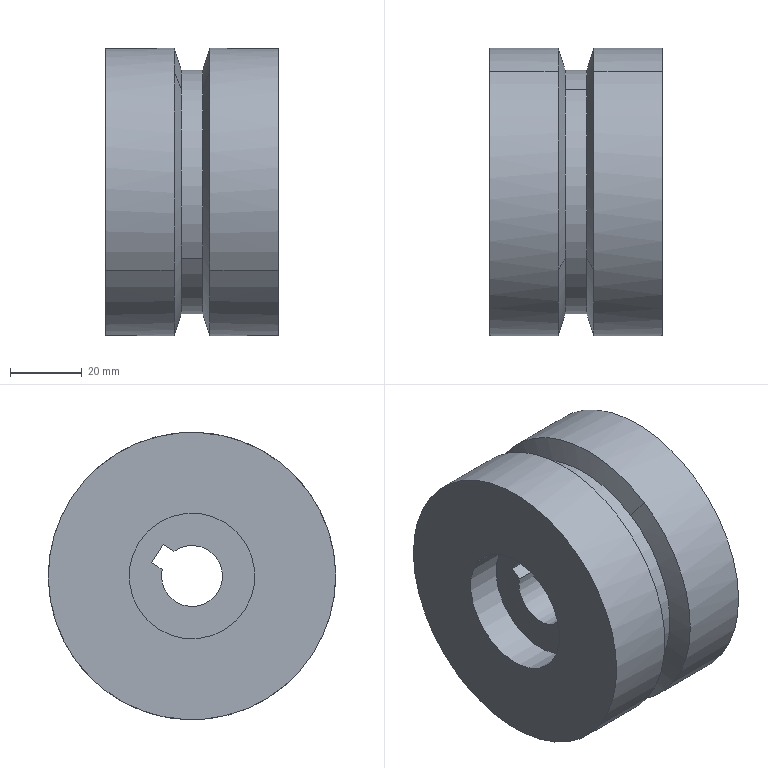Component | SolidWorks | CCD06DriveWheel-1 | 1 solid | 22 faces | box 48 x 80 x 80 mm | volume 203908 mm3 | cylinder 11 | plane 7 | cone 4 | commonest cylinder face diameters 35 x4 80 x4 68 x2 17 x1
STEP:
#1=COLOUR_RGB('',0.7922,0.8196,0.9333);
#2=FILL_AREA_STYLE_COLOUR('',#1);
#3=FILL_AREA_STYLE('',(#2));
#4=SURFACE_STYLE_FILL_AREA(#3);
#5=SURFACE_SIDE_STYLE('',(#4));
#6=SURFACE_STYLE_USAGE(.BOTH.,#5);
#7=PRESENTATION_STYLE_ASSIGNMENT((#6));
#8=CARTESIAN_POINT('',(-13.548,3.645,-4.274));
#9=VERTEX_POINT('',#8);
#10=CARTESIAN_POINT('',(-13.548,4.8,-3.522));
#11=VERTEX_POINT('',#10);
#12=CARTESIAN_POINT('',(-13.548,4.222,-3.898));
#13=DIRECTION('',(-1.,-0.,0.));
#14=DIRECTION('',(0.,0.8379,0.5458));
#15=AXIS2_PLACEMENT_3D('',#12,#13,#14);
#16=CIRCLE('',#15,0.689);
#17=EDGE_CURVE('',#9,#11,#16,.T.);
#18=ORIENTED_EDGE('',*,*,#17,.F.);
#19=CARTESIAN_POINT('',(-13.942,3.645,-4.274));
#20=VERTEX_POINT('',#19);
#21=CARTESIAN_POINT('',(-13.548,3.645,-4.274));
#22=DIRECTION('',(-1.,-0.,0.));
#23=VECTOR('',#22,39.37);
#24=LINE('',#21,#23);
#25=EDGE_CURVE('',#9,#20,#24,.T.);
#26=ORIENTED_EDGE('',*,*,#25,.T.);
#27=CARTESIAN_POINT('',(-13.942,4.8,-3.522));
#28=VERTEX_POINT('',#27);
#29=CARTESIAN_POINT('',(-13.942,4.222,-3.898));
#30=DIRECTION('',(-1.,-0.,0.));
#31=DIRECTION('',(0.,0.8379,0.5458));
#32=AXIS2_PLACEMENT_3D('',#29,#30,#31);
#33=CIRCLE('',#32,0.689);
#34=EDGE_CURVE('',#20,#28,#33,.T.);
#35=ORIENTED_EDGE('',*,*,#34,.T.);
#36=CARTESIAN_POINT('',(-13.548,4.8,-3.522));
#37=DIRECTION('',(-1.,-0.,0.));
#38=VECTOR('',#37,39.37);
#39=LINE('',#36,#38);
#40=EDGE_CURVE('',#11,#28,#39,.T.);
#41=ORIENTED_EDGE('',*,*,#40,.F.);
#42=EDGE_LOOP('',(#18,#26,#35,#41));
#43=FACE_OUTER_BOUND('',#42,.T.);
#44=CARTESIAN_POINT('',(-13.548,4.222,-3.898));
#45=DIRECTION('',(-1.,-0.,0.));
#46=DIRECTION('',(0.,0.8379,0.5458));
#47=AXIS2_PLACEMENT_3D('',#44,#45,#46);
#48=CYLINDRICAL_SURFACE('',#47,0.689);
#49=ADVANCED_FACE('',(#43),#48,.F.);
#50=CARTESIAN_POINT('',(-12.446,4.8,-3.522));
#51=VERTEX_POINT('',#50);
#52=CARTESIAN_POINT('',(-12.446,3.645,-4.274));
#53=VERTEX_POINT('',#52);
#54=CARTESIAN_POINT('',(-12.446,4.222,-3.898));
#55=DIRECTION('',(1.,0.,-0.));
#56=DIRECTION('',(-0.,-0.8379,-0.5458));
#57=AXIS2_PLACEMENT_3D('',#54,#55,#56);
#58=CIRCLE('',#57,0.689);
#59=EDGE_CURVE('',#51,#53,#58,.T.);
#60=ORIENTED_EDGE('',*,*,#59,.F.);
#61=CARTESIAN_POINT('',(-12.052,4.8,-3.522));
#62=VERTEX_POINT('',#61);
#63=CARTESIAN_POINT('',(-12.446,4.8,-3.522));
#64=DIRECTION('',(1.,0.,-0.));
#65=VECTOR('',#64,39.37);
#66=LINE('',#63,#65);
#67=EDGE_CURVE('',#51,#62,#66,.T.);
#68=ORIENTED_EDGE('',*,*,#67,.T.);
#69=CARTESIAN_POINT('',(-12.052,3.645,-4.274));
#70=VERTEX_POINT('',#69);
#71=CARTESIAN_POINT('',(-12.052,4.222,-3.898));
#72=DIRECTION('',(1.,0.,-0.));
#73=DIRECTION('',(-0.,-0.8379,-0.5458));
#74=AXIS2_PLACEMENT_3D('',#71,#72,#73);
#75=CIRCLE('',#74,0.689);
#76=EDGE_CURVE('',#62,#70,#75,.T.);
#77=ORIENTED_EDGE('',*,*,#76,.T.);
#78=CARTESIAN_POINT('',(-12.446,3.645,-4.274));
#79=DIRECTION('',(1.,0.,-0.));
#80=VECTOR('',#79,39.37);
#81=LINE('',#78,#80);
#82=EDGE_CURVE('',#53,#70,#81,.T.);
#83=ORIENTED_EDGE('',*,*,#82,.F.);
#84=EDGE_LOOP('',(#60,#68,#77,#83));
#85=FACE_OUTER_BOUND('',#84,.T.);
#86=CARTESIAN_POINT('',(-12.446,4.222,-3.898));
#87=DIRECTION('',(1.,0.,-0.));
#88=DIRECTION('',(-0.,-0.8379,-0.5458));
#89=AXIS2_PLACEMENT_3D('',#86,#87,#88);
#90=CYLINDRICAL_SURFACE('',#89,0.689);
#91=ADVANCED_FACE('',(#85),#90,.F.);
#92=CARTESIAN_POINT('',(-12.8,5.082,-5.217));
#93=VERTEX_POINT('',#92);
#94=CARTESIAN_POINT('',(-12.8,5.542,-3.038));
#95=VERTEX_POINT('',#94);
#96=CARTESIAN_POINT('',(-12.8,4.222,-3.898));
#97=DIRECTION('',(1.,0.,-0.));
#98=DIRECTION('',(-0.,-0.8379,-0.5458));
#99=AXIS2_PLACEMENT_3D('',#96,#97,#98);
#100=CIRCLE('',#99,1.575);
#101=EDGE_CURVE('',#93,#95,#100,.T.);
#102=ORIENTED_EDGE('',*,*,#101,.T.);
#103=CARTESIAN_POINT('',(-12.052,5.542,-3.038));
#104=VERTEX_POINT('',#103);
#105=CARTESIAN_POINT('',(-14.036,5.542,-3.038));
#106=DIRECTION('',(1.,0.,-0.));
#107=VECTOR('',#106,39.37);
#108=LINE('',#105,#107);
#109=EDGE_CURVE('',#95,#104,#108,.T.);
#110=ORIENTED_EDGE('',*,*,#109,.T.);
#111=CARTESIAN_POINT('',(-12.052,2.903,-4.757));
#112=VERTEX_POINT('',#111);
#113=CARTESIAN_POINT('',(-12.052,4.222,-3.898));
#114=DIRECTION('',(1.,0.,-0.));
#115=DIRECTION('',(-0.,-0.8379,-0.5458));
#116=AXIS2_PLACEMENT_3D('',#113,#114,#115);
#117=CIRCLE('',#116,1.575);
#118=EDGE_CURVE('',#112,#104,#117,.T.);
#119=ORIENTED_EDGE('',*,*,#118,.F.);
#120=CARTESIAN_POINT('',(-12.8,2.903,-4.757));
#121=VERTEX_POINT('',#120);
#122=CARTESIAN_POINT('',(-14.036,2.903,-4.757));
#123=DIRECTION('',(1.,0.,-0.));
#124=VECTOR('',#123,39.37);
#125=LINE('',#122,#124);
#126=EDGE_CURVE('',#121,#112,#125,.T.);
#127=ORIENTED_EDGE('',*,*,#126,.F.);
#128=CARTESIAN_POINT('',(-12.8,4.222,-3.898));
#129=DIRECTION('',(1.,0.,-0.));
#130=DIRECTION('',(-0.,-0.8379,-0.5458));
#131=AXIS2_PLACEMENT_3D('',#128,#129,#130);
#132=CIRCLE('',#131,1.575);
#133=EDGE_CURVE('',#121,#93,#132,.T.);
#134=ORIENTED_EDGE('',*,*,#133,.T.);
#135=EDGE_LOOP('',(#102,#110,#119,#127,#134));
#136=FACE_OUTER_BOUND('',#135,.T.);
#137=CARTESIAN_POINT('',(-14.036,4.222,-3.898));
#138=DIRECTION('',(1.,0.,-0.));
#139=DIRECTION('',(-0.,-0.8379,-0.5458));
#140=AXIS2_PLACEMENT_3D('',#137,#138,#139);
#141=CYLINDRICAL_SURFACE('',#140,1.575);
#142=ADVANCED_FACE('',(#136),#141,.T.);
#143=CARTESIAN_POINT('',(-12.879,3.101,-4.628));
#144=VERTEX_POINT('',#143);
#145=CARTESIAN_POINT('',(-12.879,4.953,-5.019));
#146=VERTEX_POINT('',#145);
#147=CARTESIAN_POINT('',(-12.879,4.222,-3.898));
#148=DIRECTION('',(1.,0.,-0.));
#149=DIRECTION('',(0.,0.8379,0.5458));
#150=AXIS2_PLACEMENT_3D('',#147,#148,#149);
#151=CIRCLE('',#150,1.339);
#152=EDGE_CURVE('',#144,#146,#151,.T.);
#153=ORIENTED_EDGE('',*,*,#152,.T.);
#154=CARTESIAN_POINT('',(-12.8,5.082,-5.217));
#155=DIRECTION('',(0.3162,0.5178,-0.7949));
#156=VECTOR('',#155,39.37);
#157=LINE('',#154,#156);
#158=EDGE_CURVE('',#146,#93,#157,.T.);
#159=ORIENTED_EDGE('',*,*,#158,.T.);
#160=ORIENTED_EDGE('',*,*,#133,.F.);
#161=CARTESIAN_POINT('',(-12.8,3.363,-2.578));
#162=VERTEX_POINT('',#161);
#163=CARTESIAN_POINT('',(-12.8,4.222,-3.898));
#164=DIRECTION('',(1.,0.,-0.));
#165=DIRECTION('',(-0.,-0.8379,-0.5458));
#166=AXIS2_PLACEMENT_3D('',#163,#164,#165);
#167=CIRCLE('',#166,1.575);
#168=EDGE_CURVE('',#162,#121,#167,.T.);
#169=ORIENTED_EDGE('',*,*,#168,.F.);
#170=CARTESIAN_POINT('',(-12.879,3.492,-2.776));
#171=VERTEX_POINT('',#170);
#172=CARTESIAN_POINT('',(-12.8,3.363,-2.578));
#173=DIRECTION('',(0.3162,-0.5178,0.7949));
#174=VECTOR('',#173,39.37);
#175=LINE('',#172,#174);
#176=EDGE_CURVE('',#171,#162,#175,.T.);
#177=ORIENTED_EDGE('',*,*,#176,.F.);
#178=CARTESIAN_POINT('',(-12.879,4.222,-3.898));
#179=DIRECTION('',(1.,0.,-0.));
#180=DIRECTION('',(0.,0.8379,0.5458));
#181=AXIS2_PLACEMENT_3D('',#178,#179,#180);
#182=CIRCLE('',#181,1.339);
#183=EDGE_CURVE('',#171,#144,#182,.T.);
#184=ORIENTED_EDGE('',*,*,#183,.T.);
#185=EDGE_LOOP('',(#153,#159,#160,#169,#177,#184));
#186=FACE_OUTER_BOUND('',#185,.T.);
#187=CARTESIAN_POINT('',(-12.8,4.222,-3.898));
#188=DIRECTION('',(1.,0.,-0.));
#189=DIRECTION('',(0.,-0.5458,0.8379));
#190=AXIS2_PLACEMENT_3D('',#187,#188,#189);
#191=CONICAL_SURFACE('',#190,1.575,1.249);
#192=ADVANCED_FACE('',(#186),#191,.T.);
#193=CARTESIAN_POINT('',(-13.942,2.903,-4.757));
#194=VERTEX_POINT('',#193);
#195=CARTESIAN_POINT('',(-13.942,5.542,-3.038));
#196=VERTEX_POINT('',#195);
#197=CARTESIAN_POINT('',(-13.942,4.222,-3.898));
#198=DIRECTION('',(1.,0.,-0.));
#199=DIRECTION('',(-0.,-0.8379,-0.5458));
#200=AXIS2_PLACEMENT_3D('',#197,#198,#199);
#201=CIRCLE('',#200,1.575);
#202=EDGE_CURVE('',#194,#196,#201,.T.);
#203=ORIENTED_EDGE('',*,*,#202,.T.);
#204=CARTESIAN_POINT('',(-13.194,5.542,-3.038));
#205=VERTEX_POINT('',#204);
#206=CARTESIAN_POINT('',(-14.036,5.542,-3.038));
#207=DIRECTION('',(1.,0.,-0.));
#208=VECTOR('',#207,39.37);
#209=LINE('',#206,#208);
#210=EDGE_CURVE('',#196,#205,#209,.T.);
#211=ORIENTED_EDGE('',*,*,#210,.T.);
#212=CARTESIAN_POINT('',(-13.194,5.082,-5.217));
#213=VERTEX_POINT('',#212);
#214=CARTESIAN_POINT('',(-13.194,4.222,-3.898));
#215=DIRECTION('',(-1.,-0.,0.));
#216=DIRECTION('',(-0.,-0.8379,-0.5458));
#217=AXIS2_PLACEMENT_3D('',#214,#215,#216);
#218=CIRCLE('',#217,1.575);
#219=EDGE_CURVE('',#205,#213,#218,.T.);
#220=ORIENTED_EDGE('',*,*,#219,.T.);
#221=CARTESIAN_POINT('',(-13.194,2.903,-4.757));
#222=VERTEX_POINT('',#221);
#223=CARTESIAN_POINT('',(-13.194,4.222,-3.898));
#224=DIRECTION('',(-1.,-0.,0.));
#225=DIRECTION('',(-0.,-0.8379,-0.5458));
#226=AXIS2_PLACEMENT_3D('',#223,#224,#225);
#227=CIRCLE('',#226,1.575);
#228=EDGE_CURVE('',#213,#222,#227,.T.);
#229=ORIENTED_EDGE('',*,*,#228,.T.);
#230=CARTESIAN_POINT('',(-14.036,2.903,-4.757));
#231=DIRECTION('',(1.,0.,-0.));
#232=VECTOR('',#231,39.37);
#233=LINE('',#230,#232);
#234=EDGE_CURVE('',#194,#222,#233,.T.);
#235=ORIENTED_EDGE('',*,*,#234,.F.);
#236=EDGE_LOOP('',(#203,#211,#220,#229,#235));
#237=FACE_OUTER_BOUND('',#236,.T.);
#238=CARTESIAN_POINT('',(-14.036,4.222,-3.898));
#239=DIRECTION('',(1.,0.,-0.));
#240=DIRECTION('',(-0.,-0.8379,-0.5458));
#241=AXIS2_PLACEMENT_3D('',#238,#239,#240);
#242=CYLINDRICAL_SURFACE('',#241,1.575);
#243=ADVANCED_FACE('',(#237),#242,.T.);
#244=CARTESIAN_POINT('',(-13.115,4.953,-5.019));
#245=VERTEX_POINT('',#244);
#246=CARTESIAN_POINT('',(-13.115,5.344,-3.167));
#247=VERTEX_POINT('',#246);
#248=CARTESIAN_POINT('',(-13.115,4.222,-3.898));
#249=DIRECTION('',(1.,0.,-0.));
#250=DIRECTION('',(-0.,-0.8379,-0.5458));
#251=AXIS2_PLACEMENT_3D('',#248,#249,#250);
#252=CIRCLE('',#251,1.339);
#253=EDGE_CURVE('',#245,#247,#252,.T.);
#254=ORIENTED_EDGE('',*,*,#253,.T.);
#255=CARTESIAN_POINT('',(-12.879,5.344,-3.167));
#256=VERTEX_POINT('',#255);
#257=CARTESIAN_POINT('',(-14.036,5.344,-3.167));
#258=DIRECTION('',(1.,0.,-0.));
#259=VECTOR('',#258,39.37);
#260=LINE('',#257,#259);
#261=EDGE_CURVE('',#247,#256,#260,.T.);
#262=ORIENTED_EDGE('',*,*,#261,.T.);
#263=CARTESIAN_POINT('',(-12.879,4.222,-3.898));
#264=DIRECTION('',(1.,0.,-0.));
#265=DIRECTION('',(0.,0.8379,0.5458));
#266=AXIS2_PLACEMENT_3D('',#263,#264,#265);
#267=CIRCLE('',#266,1.339);
#268=EDGE_CURVE('',#146,#256,#267,.T.);
#269=ORIENTED_EDGE('',*,*,#268,.F.);
#270=ORIENTED_EDGE('',*,*,#152,.F.);
#271=CARTESIAN_POINT('',(-13.115,3.101,-4.628));
#272=VERTEX_POINT('',#271);
#273=CARTESIAN_POINT('',(-14.036,3.101,-4.628));
#274=DIRECTION('',(1.,0.,-0.));
#275=VECTOR('',#274,39.37);
#276=LINE('',#273,#275);
#277=EDGE_CURVE('',#272,#144,#276,.T.);
#278=ORIENTED_EDGE('',*,*,#277,.F.);
#279=CARTESIAN_POINT('',(-13.115,4.222,-3.898));
#280=DIRECTION('',(1.,0.,-0.));
#281=DIRECTION('',(-0.,-0.8379,-0.5458));
#282=AXIS2_PLACEMENT_3D('',#279,#280,#281);
#283=CIRCLE('',#282,1.339);
#284=EDGE_CURVE('',#272,#245,#283,.T.);
#285=ORIENTED_EDGE('',*,*,#284,.T.);
#286=EDGE_LOOP('',(#254,#262,#269,#270,#278,#285));
#287=FACE_OUTER_BOUND('',#286,.T.);
#288=CARTESIAN_POINT('',(-14.036,4.222,-3.898));
#289=DIRECTION('',(1.,0.,-0.));
#290=DIRECTION('',(-0.,-0.8379,-0.5458));
#291=AXIS2_PLACEMENT_3D('',#288,#289,#290);
#292=CYLINDRICAL_SURFACE('',#291,1.339);
#293=ADVANCED_FACE('',(#287),#292,.T.);
#294=CARTESIAN_POINT('',(-13.115,3.492,-2.776));
#295=VERTEX_POINT('',#294);
#296=CARTESIAN_POINT('',(-13.115,4.222,-3.898));
#297=DIRECTION('',(1.,0.,-0.));
#298=DIRECTION('',(-0.,-0.8379,-0.5458));
#299=AXIS2_PLACEMENT_3D('',#296,#297,#298);
#300=CIRCLE('',#299,1.339);
#301=EDGE_CURVE('',#295,#272,#300,.T.);
#302=ORIENTED_EDGE('',*,*,#301,.F.);
#303=CARTESIAN_POINT('',(-13.194,3.363,-2.578));
#304=VERTEX_POINT('',#303);
#305=CARTESIAN_POINT('',(-13.194,3.363,-2.578));
#306=DIRECTION('',(-0.3162,-0.5178,0.7949));
#307=VECTOR('',#306,39.37);
#308=LINE('',#305,#307);
#309=EDGE_CURVE('',#295,#304,#308,.T.);
#310=ORIENTED_EDGE('',*,*,#309,.T.);
#311=CARTESIAN_POINT('',(-13.194,4.222,-3.898));
#312=DIRECTION('',(-1.,-0.,0.));
#313=DIRECTION('',(-0.,-0.8379,-0.5458));
#314=AXIS2_PLACEMENT_3D('',#311,#312,#313);
#315=CIRCLE('',#314,1.575);
#316=EDGE_CURVE('',#222,#304,#315,.T.);
#317=ORIENTED_EDGE('',*,*,#316,.F.);
#318=ORIENTED_EDGE('',*,*,#228,.F.);
#319=CARTESIAN_POINT('',(-13.194,5.082,-5.217));
#320=DIRECTION('',(-0.3162,0.5178,-0.7949));
#321=VECTOR('',#320,39.37);
#322=LINE('',#319,#321);
#323=EDGE_CURVE('',#245,#213,#322,.T.);
#324=ORIENTED_EDGE('',*,*,#323,.F.);
#325=ORIENTED_EDGE('',*,*,#284,.F.);
#326=EDGE_LOOP('',(#302,#310,#317,#318,#324,#325));
#327=FACE_OUTER_BOUND('',#326,.T.);
#328=CARTESIAN_POINT('',(-13.194,4.222,-3.898));
#329=DIRECTION('',(-1.,-0.,0.));
#330=DIRECTION('',(-0.,0.5458,-0.8379));
#331=AXIS2_PLACEMENT_3D('',#328,#329,#330);
#332=CONICAL_SURFACE('',#331,1.575,1.249);
#333=ADVANCED_FACE('',(#327),#332,.T.);
#334=CARTESIAN_POINT('',(-13.548,4.42,-3.628));
#335=VERTEX_POINT('',#334);
#336=CARTESIAN_POINT('',(-13.548,4.549,-3.826));
#337=VERTEX_POINT('',#336);
#338=CARTESIAN_POINT('',(-13.548,4.222,-3.898));
#339=DIRECTION('',(1.,0.,-0.));
#340=DIRECTION('',(0.,0.8379,0.5458));
#341=AXIS2_PLACEMENT_3D('',#338,#339,#340);
#342=CIRCLE('',#341,0.3346);
#343=EDGE_CURVE('',#335,#337,#342,.T.);
#344=ORIENTED_EDGE('',*,*,#343,.F.);
#345=CARTESIAN_POINT('',(-12.446,4.42,-3.628));
#346=VERTEX_POINT('',#345);
#347=CARTESIAN_POINT('',(-13.942,4.42,-3.628));
#348=DIRECTION('',(1.,0.,-0.));
#349=VECTOR('',#348,39.37);
#350=LINE('',#347,#349);
#351=EDGE_CURVE('',#335,#346,#350,.T.);
#352=ORIENTED_EDGE('',*,*,#351,.T.);
#353=CARTESIAN_POINT('',(-12.446,4.549,-3.826));
#354=VERTEX_POINT('',#353);
#355=CARTESIAN_POINT('',(-12.446,4.222,-3.898));
#356=DIRECTION('',(-1.,-0.,0.));
#357=DIRECTION('',(0.,-0.8379,-0.5458));
#358=AXIS2_PLACEMENT_3D('',#355,#356,#357);
#359=CIRCLE('',#358,0.3346);
#360=EDGE_CURVE('',#354,#346,#359,.T.);
#361=ORIENTED_EDGE('',*,*,#360,.F.);
#362=CARTESIAN_POINT('',(-13.942,4.549,-3.826));
#363=DIRECTION('',(-1.,-0.,0.));
#364=VECTOR('',#363,39.37);
#365=LINE('',#362,#364);
#366=EDGE_CURVE('',#354,#337,#365,.T.);
#367=ORIENTED_EDGE('',*,*,#366,.T.);
#368=EDGE_LOOP('',(#344,#352,#361,#367));
#369=FACE_OUTER_BOUND('',#368,.T.);
#370=CARTESIAN_POINT('',(-13.942,4.222,-3.898));
#371=DIRECTION('',(-1.,-0.,0.));
#372=DIRECTION('',(0.,0.8379,0.5458));
#373=AXIS2_PLACEMENT_3D('',#370,#371,#372);
#374=CYLINDRICAL_SURFACE('',#373,0.3346);
#375=ADVANCED_FACE('',(#369),#374,.F.);
#376=CARTESIAN_POINT('',(-13.548,4.537,-3.552));
#377=VERTEX_POINT('',#376);
#378=CARTESIAN_POINT('',(-13.548,4.42,-3.628));
#379=DIRECTION('',(-0.,-0.8379,-0.5458));
#380=VECTOR('',#379,39.37);
#381=LINE('',#378,#380);
#382=EDGE_CURVE('',#377,#335,#381,.T.);
#383=ORIENTED_EDGE('',*,*,#382,.F.);
#384=CARTESIAN_POINT('',(-12.446,4.537,-3.552));
#385=VERTEX_POINT('',#384);
#386=CARTESIAN_POINT('',(-13.942,4.537,-3.552));
#387=DIRECTION('',(1.,0.,-0.));
#388=VECTOR('',#387,39.37);
#389=LINE('',#386,#388);
#390=EDGE_CURVE('',#377,#385,#389,.T.);
#391=ORIENTED_EDGE('',*,*,#390,.T.);
#392=CARTESIAN_POINT('',(-12.446,4.42,-3.628));
#393=DIRECTION('',(0.,0.8379,0.5458));
#394=VECTOR('',#393,39.37);
#395=LINE('',#392,#394);
#396=EDGE_CURVE('',#346,#385,#395,.T.);
#397=ORIENTED_EDGE('',*,*,#396,.F.);
#398=ORIENTED_EDGE('',*,*,#351,.F.);
#399=EDGE_LOOP('',(#383,#391,#397,#398));
#400=FACE_OUTER_BOUND('',#399,.T.);
#401=CARTESIAN_POINT('',(-13.942,4.42,-3.628));
#402=DIRECTION('',(0.,-0.5458,0.8379));
#403=DIRECTION('',(-1.,-0.,0.));
#404=AXIS2_PLACEMENT_3D('',#401,#402,#403);
#405=PLANE('',#404);
#406=ADVANCED_FACE('',(#400),#405,.F.);
#407=CARTESIAN_POINT('',(-13.548,4.666,-3.749));
#408=VERTEX_POINT('',#407);
#409=CARTESIAN_POINT('',(-13.548,4.537,-3.552));
#410=DIRECTION('',(0.,-0.5458,0.8379));
#411=VECTOR('',#410,39.37);
#412=LINE('',#409,#411);
#413=EDGE_CURVE('',#408,#377,#412,.T.);
#414=ORIENTED_EDGE('',*,*,#413,.F.);
#415=CARTESIAN_POINT('',(-12.446,4.666,-3.749));
#416=VERTEX_POINT('',#415);
#417=CARTESIAN_POINT('',(-13.942,4.666,-3.749));
#418=DIRECTION('',(1.,0.,-0.));
#419=VECTOR('',#418,39.37);
#420=LINE('',#417,#419);
#421=EDGE_CURVE('',#408,#416,#420,.T.);
#422=ORIENTED_EDGE('',*,*,#421,.T.);
#423=CARTESIAN_POINT('',(-12.446,4.537,-3.552));
#424=DIRECTION('',(-0.,0.5458,-0.8379));
#425=VECTOR('',#424,39.37);
#426=LINE('',#423,#425);
#427=EDGE_CURVE('',#385,#416,#426,.T.);
#428=ORIENTED_EDGE('',*,*,#427,.F.);
#429=ORIENTED_EDGE('',*,*,#390,.F.);
#430=EDGE_LOOP('',(#414,#422,#428,#429));
#431=FACE_OUTER_BOUND('',#430,.T.);
#432=CARTESIAN_POINT('',(-13.942,4.537,-3.552));
#433=DIRECTION('',(0.,0.8379,0.5458));
#434=DIRECTION('',(1.,0.,-0.));
#435=AXIS2_PLACEMENT_3D('',#432,#433,#434);
#436=PLANE('',#435);
#437=ADVANCED_FACE('',(#431),#436,.F.);
#438=CARTESIAN_POINT('',(-13.548,4.666,-3.749));
#439=DIRECTION('',(0.,0.8379,0.5458));
#440=VECTOR('',#439,39.37);
#441=LINE('',#438,#440);
#442=EDGE_CURVE('',#337,#408,#441,.T.);
#443=ORIENTED_EDGE('',*,*,#442,.F.);
#444=ORIENTED_EDGE('',*,*,#366,.F.);
#445=CARTESIAN_POINT('',(-12.446,4.666,-3.749));
#446=DIRECTION('',(-0.,-0.8379,-0.5458));
#447=VECTOR('',#446,39.37);
#448=LINE('',#445,#447);
#449=EDGE_CURVE('',#416,#354,#448,.T.);
#450=ORIENTED_EDGE('',*,*,#449,.F.);
#451=ORIENTED_EDGE('',*,*,#421,.F.);
#452=EDGE_LOOP('',(#443,#444,#450,#451));
#453=FACE_OUTER_BOUND('',#452,.T.);
#454=CARTESIAN_POINT('',(-13.942,4.666,-3.749));
#455=DIRECTION('',(-0.,0.5458,-0.8379));
#456=DIRECTION('',(1.,0.,-0.));
#457=AXIS2_PLACEMENT_3D('',#454,#455,#456);
#458=PLANE('',#457);
#459=ADVANCED_FACE('',(#453),#458,.F.);
#460=CARTESIAN_POINT('',(-12.052,4.222,-3.898));
#461=DIRECTION('',(1.,0.,-0.));
#462=DIRECTION('',(-0.,-0.8379,-0.5458));
#463=AXIS2_PLACEMENT_3D('',#460,#461,#462);
#464=CIRCLE('',#463,0.689);
#465=EDGE_CURVE('',#70,#62,#464,.T.);
#466=ORIENTED_EDGE('',*,*,#465,.F.);
#467=ORIENTED_EDGE('',*,*,#76,.F.);
#468=EDGE_LOOP('',(#466,#467));
#469=FACE_BOUND('',#468,.T.);
#470=ORIENTED_EDGE('',*,*,#118,.T.);
#471=CARTESIAN_POINT('',(-12.052,4.222,-3.898));
#472=DIRECTION('',(1.,0.,-0.));
#473=DIRECTION('',(-0.,-0.8379,-0.5458));
#474=AXIS2_PLACEMENT_3D('',#471,#472,#473);
#475=CIRCLE('',#474,1.575);
#476=EDGE_CURVE('',#104,#112,#475,.T.);
#477=ORIENTED_EDGE('',*,*,#476,.T.);
#478=EDGE_LOOP('',(#470,#477));
#479=FACE_OUTER_BOUND('',#478,.T.);
#480=CARTESIAN_POINT('',(-12.052,4.222,-3.898));
#481=DIRECTION('',(1.,0.,-0.));
#482=DIRECTION('',(-0.,-0.8379,-0.5458));
#483=AXIS2_PLACEMENT_3D('',#480,#481,#482);
#484=PLANE('',#483);
#485=ADVANCED_FACE('',(#469,#479),#484,.T.);
#486=ORIENTED_EDGE('',*,*,#109,.F.);
#487=CARTESIAN_POINT('',(-12.8,4.222,-3.898));
#488=DIRECTION('',(1.,0.,-0.));
#489=DIRECTION('',(-0.,-0.8379,-0.5458));
#490=AXIS2_PLACEMENT_3D('',#487,#488,#489);
#491=CIRCLE('',#490,1.575);
#492=EDGE_CURVE('',#95,#162,#491,.T.);
#493=ORIENTED_EDGE('',*,*,#492,.T.);
#494=ORIENTED_EDGE('',*,*,#168,.T.);
#495=ORIENTED_EDGE('',*,*,#126,.T.);
#496=ORIENTED_EDGE('',*,*,#476,.F.);
#497=EDGE_LOOP('',(#486,#493,#494,#495,#496));
#498=FACE_OUTER_BOUND('',#497,.T.);
#499=CARTESIAN_POINT('',(-14.036,4.222,-3.898));
#500=DIRECTION('',(1.,0.,-0.));
#501=DIRECTION('',(-0.,-0.8379,-0.5458));
#502=AXIS2_PLACEMENT_3D('',#499,#500,#501);
#503=CYLINDRICAL_SURFACE('',#502,1.575);
#504=ADVANCED_FACE('',(#498),#503,.T.);
#505=CARTESIAN_POINT('',(-13.942,4.222,-3.898));
#506=DIRECTION('',(-1.,-0.,0.));
#507=DIRECTION('',(0.,0.8379,0.5458));
#508=AXIS2_PLACEMENT_3D('',#505,#506,#507);
#509=CIRCLE('',#508,0.689);
#510=EDGE_CURVE('',#28,#20,#509,.T.);
#511=ORIENTED_EDGE('',*,*,#510,.F.);
#512=ORIENTED_EDGE('',*,*,#34,.F.);
#513=EDGE_LOOP('',(#511,#512));
#514=FACE_BOUND('',#513,.T.);
#515=ORIENTED_EDGE('',*,*,#202,.F.);
#516=CARTESIAN_POINT('',(-13.942,4.222,-3.898));
#517=DIRECTION('',(1.,0.,-0.));
#518=DIRECTION('',(-0.,-0.8379,-0.5458));
#519=AXIS2_PLACEMENT_3D('',#516,#517,#518);
#520=CIRCLE('',#519,1.575);
#521=EDGE_CURVE('',#196,#194,#520,.T.);
#522=ORIENTED_EDGE('',*,*,#521,.F.);
#523=EDGE_LOOP('',(#515,#522));
#524=FACE_OUTER_BOUND('',#523,.T.);
#525=CARTESIAN_POINT('',(-13.942,4.222,-3.898));
#526=DIRECTION('',(1.,0.,-0.));
#527=DIRECTION('',(-0.,-0.8379,-0.5458));
#528=AXIS2_PLACEMENT_3D('',#525,#526,#527);
#529=PLANE('',#528);
#530=ADVANCED_FACE('',(#514,#524),#529,.F.);
#531=ORIENTED_EDGE('',*,*,#158,.F.);
#532=ORIENTED_EDGE('',*,*,#268,.T.);
#533=CARTESIAN_POINT('',(-12.879,4.222,-3.898));
#534=DIRECTION('',(1.,0.,-0.));
#535=DIRECTION('',(0.,0.8379,0.5458));
#536=AXIS2_PLACEMENT_3D('',#533,#534,#535);
#537=CIRCLE('',#536,1.339);
#538=EDGE_CURVE('',#256,#171,#537,.T.);
#539=ORIENTED_EDGE('',*,*,#538,.T.);
#540=ORIENTED_EDGE('',*,*,#176,.T.);
#541=ORIENTED_EDGE('',*,*,#492,.F.);
#542=ORIENTED_EDGE('',*,*,#101,.F.);
#543=EDGE_LOOP('',(#531,#532,#539,#540,#541,#542));
#544=FACE_OUTER_BOUND('',#543,.T.);
#545=CARTESIAN_POINT('',(-12.8,4.222,-3.898));
#546=DIRECTION('',(1.,0.,-0.));
#547=DIRECTION('',(0.,-0.5458,0.8379));
#548=AXIS2_PLACEMENT_3D('',#545,#546,#547);
#549=CONICAL_SURFACE('',#548,1.575,1.249);
#550=ADVANCED_FACE('',(#544),#549,.T.);
#551=ORIENTED_EDGE('',*,*,#210,.F.);
#552=ORIENTED_EDGE('',*,*,#521,.T.);
#553=ORIENTED_EDGE('',*,*,#234,.T.);
#554=ORIENTED_EDGE('',*,*,#316,.T.);
#555=CARTESIAN_POINT('',(-13.194,4.222,-3.898));
#556=DIRECTION('',(-1.,-0.,0.));
#557=DIRECTION('',(-0.,-0.8379,-0.5458));
#558=AXIS2_PLACEMENT_3D('',#555,#556,#557);
#559=CIRCLE('',#558,1.575);
#560=EDGE_CURVE('',#304,#205,#559,.T.);
#561=ORIENTED_EDGE('',*,*,#560,.T.);
#562=EDGE_LOOP('',(#551,#552,#553,#554,#561));
#563=FACE_OUTER_BOUND('',#562,.T.);
#564=CARTESIAN_POINT('',(-14.036,4.222,-3.898));
#565=DIRECTION('',(1.,0.,-0.));
#566=DIRECTION('',(-0.,-0.8379,-0.5458));
#567=AXIS2_PLACEMENT_3D('',#564,#565,#566);
#568=CYLINDRICAL_SURFACE('',#567,1.575);
#569=ADVANCED_FACE('',(#563),#568,.T.);
#570=ORIENTED_EDGE('',*,*,#261,.F.);
#571=CARTESIAN_POINT('',(-13.115,4.222,-3.898));
#572=DIRECTION('',(1.,0.,-0.));
#573=DIRECTION('',(-0.,-0.8379,-0.5458));
#574=AXIS2_PLACEMENT_3D('',#571,#572,#573);
#575=CIRCLE('',#574,1.339);
#576=EDGE_CURVE('',#247,#295,#575,.T.);
#577=ORIENTED_EDGE('',*,*,#576,.T.);
#578=ORIENTED_EDGE('',*,*,#301,.T.);
#579=ORIENTED_EDGE('',*,*,#277,.T.);
#580=ORIENTED_EDGE('',*,*,#183,.F.);
#581=ORIENTED_EDGE('',*,*,#538,.F.);
#582=EDGE_LOOP('',(#570,#577,#578,#579,#580,#581));
#583=FACE_OUTER_BOUND('',#582,.T.);
#584=CARTESIAN_POINT('',(-14.036,4.222,-3.898));
#585=DIRECTION('',(1.,0.,-0.));
#586=DIRECTION('',(-0.,-0.8379,-0.5458));
#587=AXIS2_PLACEMENT_3D('',#584,#585,#586);
#588=CYLINDRICAL_SURFACE('',#587,1.339);
#589=ADVANCED_FACE('',(#583),#588,.T.);
#590=ORIENTED_EDGE('',*,*,#309,.F.);
#591=ORIENTED_EDGE('',*,*,#576,.F.);
#592=ORIENTED_EDGE('',*,*,#253,.F.);
#593=ORIENTED_EDGE('',*,*,#323,.T.);
#594=ORIENTED_EDGE('',*,*,#219,.F.);
#595=ORIENTED_EDGE('',*,*,#560,.F.);
#596=EDGE_LOOP('',(#590,#591,#592,#593,#594,#595));
#597=FACE_OUTER_BOUND('',#596,.T.);
#598=CARTESIAN_POINT('',(-13.194,4.222,-3.898));
#599=DIRECTION('',(-1.,-0.,0.));
#600=DIRECTION('',(-0.,0.5458,-0.8379));
#601=AXIS2_PLACEMENT_3D('',#598,#599,#600);
#602=CONICAL_SURFACE('',#601,1.575,1.249);
#603=ADVANCED_FACE('',(#597),#602,.T.);
#604=CARTESIAN_POINT('',(-12.446,4.222,-3.898));
#605=DIRECTION('',(1.,0.,-0.));
#606=DIRECTION('',(-0.,-0.8379,-0.5458));
#607=AXIS2_PLACEMENT_3D('',#604,#605,#606);
#608=CIRCLE('',#607,0.689);
#609=EDGE_CURVE('',#53,#51,#608,.T.);
#610=ORIENTED_EDGE('',*,*,#609,.T.);
#611=ORIENTED_EDGE('',*,*,#59,.T.);
#612=EDGE_LOOP('',(#610,#611));
#613=FACE_OUTER_BOUND('',#612,.T.);
#614=ORIENTED_EDGE('',*,*,#360,.T.);
#615=ORIENTED_EDGE('',*,*,#396,.T.);
#616=ORIENTED_EDGE('',*,*,#427,.T.);
#617=ORIENTED_EDGE('',*,*,#449,.T.);
#618=EDGE_LOOP('',(#614,#615,#616,#617));
#619=FACE_BOUND('',#618,.T.);
#620=CARTESIAN_POINT('',(-12.446,4.222,-3.898));
#621=DIRECTION('',(1.,0.,-0.));
#622=DIRECTION('',(-0.,-0.8379,-0.5458));
#623=AXIS2_PLACEMENT_3D('',#620,#621,#622);
#624=PLANE('',#623);
#625=ADVANCED_FACE('',(#613,#619),#624,.T.);
#626=ORIENTED_EDGE('',*,*,#67,.F.);
#627=ORIENTED_EDGE('',*,*,#609,.F.);
#628=ORIENTED_EDGE('',*,*,#82,.T.);
#629=ORIENTED_EDGE('',*,*,#465,.T.);
#630=EDGE_LOOP('',(#626,#627,#628,#629));
#631=FACE_OUTER_BOUND('',#630,.T.);
#632=CARTESIAN_POINT('',(-12.446,4.222,-3.898));
#633=DIRECTION('',(1.,0.,-0.));
#634=DIRECTION('',(-0.,-0.8379,-0.5458));
#635=AXIS2_PLACEMENT_3D('',#632,#633,#634);
#636=CYLINDRICAL_SURFACE('',#635,0.689);
#637=ADVANCED_FACE('',(#631),#636,.F.);
#638=CARTESIAN_POINT('',(-13.548,4.222,-3.898));
#639=DIRECTION('',(-1.,-0.,0.));
#640=DIRECTION('',(0.,0.8379,0.5458));
#641=AXIS2_PLACEMENT_3D('',#638,#639,#640);
#642=CIRCLE('',#641,0.689);
#643=EDGE_CURVE('',#11,#9,#642,.T.);
#644=ORIENTED_EDGE('',*,*,#643,.T.);
#645=ORIENTED_EDGE('',*,*,#17,.T.);
#646=EDGE_LOOP('',(#644,#645));
#647=FACE_OUTER_BOUND('',#646,.T.);
#648=ORIENTED_EDGE('',*,*,#343,.T.);
#649=ORIENTED_EDGE('',*,*,#442,.T.);
#650=ORIENTED_EDGE('',*,*,#413,.T.);
#651=ORIENTED_EDGE('',*,*,#382,.T.);
#652=EDGE_LOOP('',(#648,#649,#650,#651));
#653=FACE_BOUND('',#652,.T.);
#654=CARTESIAN_POINT('',(-13.548,4.222,-3.898));
#655=DIRECTION('',(-1.,-0.,0.));
#656=DIRECTION('',(0.,0.8379,0.5458));
#657=AXIS2_PLACEMENT_3D('',#654,#655,#656);
#658=PLANE('',#657);
#659=ADVANCED_FACE('',(#647,#653),#658,.T.);
#660=ORIENTED_EDGE('',*,*,#25,.F.);
#661=ORIENTED_EDGE('',*,*,#643,.F.);
#662=ORIENTED_EDGE('',*,*,#40,.T.);
#663=ORIENTED_EDGE('',*,*,#510,.T.);
#664=EDGE_LOOP('',(#660,#661,#662,#663));
#665=FACE_OUTER_BOUND('',#664,.T.);
#666=CARTESIAN_POINT('',(-13.548,4.222,-3.898));
#667=DIRECTION('',(-1.,-0.,0.));
#668=DIRECTION('',(0.,0.8379,0.5458));
#669=AXIS2_PLACEMENT_3D('',#666,#667,#668);
#670=CYLINDRICAL_SURFACE('',#669,0.689);
#671=ADVANCED_FACE('',(#665),#670,.F.);
#672=CLOSED_SHELL('',(#49,#91,#142,#192,#243,#293,#333,#375,#406,#437,#459,#485,#504,#530,#550,#569,#589,#603,#625,#637,#659,#671));
#673=MANIFOLD_SOLID_BREP('',#672);
#674=STYLED_ITEM('',(#7),#673);
#675=PRESENTATION_LAYER_ASSIGNMENT('','',(#674));
#676=CARTESIAN_POINT('',(0.,0.,0.));
#677=DIRECTION('',(0.,0.,1.));
#678=DIRECTION('',(1.,0.,0.));
#679=AXIS2_PLACEMENT_3D('',#676,#677,#678);
#680=(LENGTH_UNIT()NAMED_UNIT(*)SI_UNIT($,.METRE.));
#681=LENGTH_MEASURE_WITH_UNIT(LENGTH_MEASURE(0.0254),#680);
#682=DIMENSIONAL_EXPONENTS(1.,0.,0.,0.,0.,0.,0.);
#683=(CONVERSION_BASED_UNIT('',#681)LENGTH_UNIT()NAMED_UNIT(#682));
#684=UNCERTAINTY_MEASURE_WITH_UNIT(LENGTH_MEASURE(0.00001),#683,'','');
#685=(NAMED_UNIT(*)PLANE_ANGLE_UNIT()SI_UNIT($,.RADIAN.));
#686=(NAMED_UNIT(*)SI_UNIT($,.STERADIAN.)SOLID_ANGLE_UNIT());
#687=(GEOMETRIC_REPRESENTATION_CONTEXT(3)GLOBAL_UNCERTAINTY_ASSIGNED_CONTEXT((#684))GLOBAL_UNIT_ASSIGNED_CONTEXT((#683,#685,#686))REPRESENTATION_CONTEXT('',''));
#688=ADVANCED_BREP_SHAPE_REPRESENTATION('',(#673,#679),#687);
#689=(LENGTH_UNIT()NAMED_UNIT(*)SI_UNIT($,.METRE.));
#690=LENGTH_MEASURE_WITH_UNIT(LENGTH_MEASURE(0.0254),#689);
#691=DIMENSIONAL_EXPONENTS(1.,0.,0.,0.,0.,0.,0.);
#692=(CONVERSION_BASED_UNIT('',#690)LENGTH_UNIT()NAMED_UNIT(#691));
#693=UNCERTAINTY_MEASURE_WITH_UNIT(LENGTH_MEASURE(0.00001),#692,'','');
#694=(NAMED_UNIT(*)PLANE_ANGLE_UNIT()SI_UNIT($,.RADIAN.));
#695=(NAMED_UNIT(*)SI_UNIT($,.STERADIAN.)SOLID_ANGLE_UNIT());
#696=(GEOMETRIC_REPRESENTATION_CONTEXT(3)GLOBAL_UNCERTAINTY_ASSIGNED_CONTEXT((#693))GLOBAL_UNIT_ASSIGNED_CONTEXT((#692,#694,#695))REPRESENTATION_CONTEXT('',''));
#697=MECHANICAL_DESIGN_GEOMETRIC_PRESENTATION_REPRESENTATION('',(#674),#696);